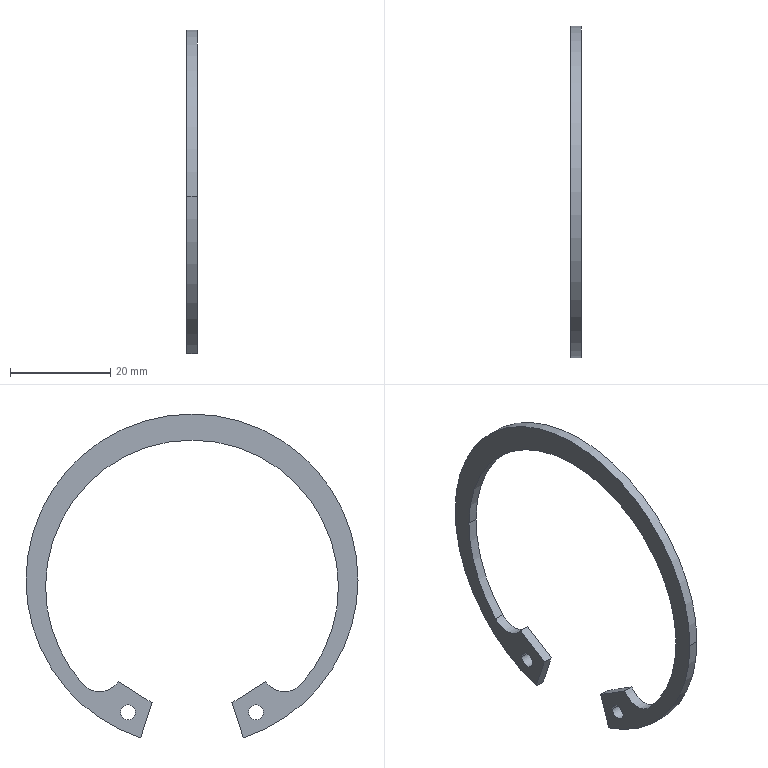Component | SolidWorks | GuideWheelAssembly-1_GB893.2-86RetainingRingForHolesTypeB62-1 | 1 solid | 18 faces | box 2 x 66.2 x 64.58 mm | volume 1598 mm3 | cylinder 12 | plane 6 | commonest cylinder face diameters 3 x4 58.4 x3 66.2 x3 8.8 x2
build123d program:
from build123d import *

# Parameters (mm, degrees)
BASE_EXTRUDE_DEPTH      = 1
BASE_EXTRUDE_DEPTH_BACK = 1
SKETCH1_R               = 1.5


with BuildPart() as part:
    # Sketch1 → Base-Extrude (new, two sides: drawn at the far end of the back side and taken through both)
    with BuildSketch(Plane.XY.offset(-BASE_EXTRUDE_DEPTH_BACK)):
        with BuildLine():
            Line((-14.724, -20.223), (-7.957, -24.49))
            Line((-7.957, -24.49), (-10.228, -31.48))
            ThreePointArc((-10.228, -31.48), (0, 33.1), (10.228, -31.48))
            Line((10.228, -31.48), (7.957, -24.49))
            Line((7.957, -24.49), (14.724, -20.223))
            ThreePointArc((14.724, -20.223), (18.074, -22.26), (21.719, -20.817))
            ThreePointArc((21.719, -20.817), (0, 27.9), (-21.719, -20.817))
            ThreePointArc((-21.719, -20.817), (-18.074, -22.26), (-14.724, -20.223))
        make_face()
        with Locations((-12.774, -26.369)):
            Circle(SKETCH1_R, mode=Mode.SUBTRACT)
        with Locations(Location((12.774, -26.369, 0), (0, 0, 180))):
            Circle(SKETCH1_R, mode=Mode.SUBTRACT)
    extrude(amount=BASE_EXTRUDE_DEPTH + BASE_EXTRUDE_DEPTH_BACK)


solid = part.part

# Placed as in the assembly
solid = solid.moved(Location((-565, 0, 25), (90, -90, 0)))